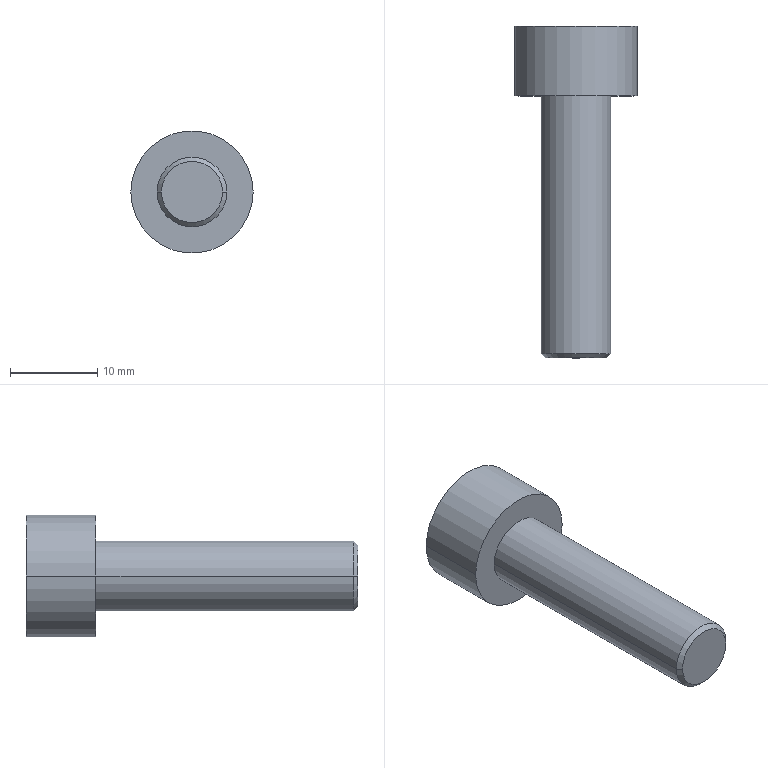Component | SolidWorks | M8x30HexSocketCap-2 | 1 solid | 16 faces | box 14 x 38 x 14 mm | volume 2553 mm3 | plane 10 | cylinder 4 | cone 2 | commonest cylinder face diameters 8 x2 14 x2 | material #45
build123d program:
from build123d import *

# Parameters (mm, degrees)
CUT_EXTRUDE1_DEPTH = 5.5


with BuildPart() as part:
    # Sketch1 → Revolve1 (revolve)
    with BuildSketch(Plane(origin=(0, 0, 0), x_dir=(1, 0, 0), z_dir=(0, 1, 0)), mode=Mode.PRIVATE) as revolve1_sk:
        Polygon((0, 38), (-7, 38), (-7, 30), (-4, 30), (-4, 0.5), (-3.5, 0), (0, 0), align=None)
    revolve(revolve1_sk.sketch.rotate(Axis((0, 0, 0), (0, 0, -1)), 180), axis=Axis((0, 0, 0), (0, 0, -1)))

    # Sketch2 → Cut-Extrude1 (cut)
    with BuildSketch(Plane(origin=(0, 0, -38), x_dir=(-1, 0, 0), z_dir=(0, 0, -1))):
        Polygon((0, 3.58), (-3.1, 1.79), (-3.1, -1.79), (0, -3.58), (3.1, -1.79), (3.1, 1.79), align=None)
    extrude(amount=-CUT_EXTRUDE1_DEPTH, mode=Mode.SUBTRACT)


solid = part.part

# Placed as in the assembly
solid = solid.moved(Location((7, -20, -15), (90, 0, 0)))
STEP:
#1=CARTESIAN_POINT('',(0.4134,-0.7874,-0.5906));
#2=VERTEX_POINT('',#1);
#3=CARTESIAN_POINT('',(0.1378,-0.7874,-0.5906));
#4=VERTEX_POINT('',#3);
#5=CARTESIAN_POINT('',(0.2756,-0.7874,-0.5906));
#6=DIRECTION('',(0.,-1.,0.));
#7=DIRECTION('',(1.,0.,0.));
#8=AXIS2_PLACEMENT_3D('',#5,#6,#7);
#9=CIRCLE('',#8,0.1378);
#10=EDGE_CURVE('',#2,#4,#9,.T.);
#11=ORIENTED_EDGE('',*,*,#10,.F.);
#12=CARTESIAN_POINT('',(0.4331,-0.7677,-0.5906));
#13=VERTEX_POINT('',#12);
#14=CARTESIAN_POINT('',(0.4331,-0.7677,-0.5906));
#15=DIRECTION('',(0.7071,0.7071,0.));
#16=VECTOR('',#15,39.37);
#17=LINE('',#14,#16);
#18=EDGE_CURVE('',#2,#13,#17,.T.);
#19=ORIENTED_EDGE('',*,*,#18,.T.);
#20=CARTESIAN_POINT('',(0.1181,-0.7677,-0.5906));
#21=VERTEX_POINT('',#20);
#22=CARTESIAN_POINT('',(0.2756,-0.7677,-0.5906));
#23=DIRECTION('',(0.,-1.,0.));
#24=DIRECTION('',(1.,0.,0.));
#25=AXIS2_PLACEMENT_3D('',#22,#23,#24);
#26=CIRCLE('',#25,0.1575);
#27=EDGE_CURVE('',#13,#21,#26,.T.);
#28=ORIENTED_EDGE('',*,*,#27,.T.);
#29=CARTESIAN_POINT('',(0.1181,-0.7677,-0.5906));
#30=DIRECTION('',(-0.7071,0.7071,0.));
#31=VECTOR('',#30,39.37);
#32=LINE('',#29,#31);
#33=EDGE_CURVE('',#4,#21,#32,.T.);
#34=ORIENTED_EDGE('',*,*,#33,.F.);
#35=EDGE_LOOP('',(#11,#19,#28,#34));
#36=FACE_OUTER_BOUND('',#35,.T.);
#37=CARTESIAN_POINT('',(0.2756,-0.7677,-0.5906));
#38=DIRECTION('',(0.,1.,0.));
#39=DIRECTION('',(-1.,0.,0.));
#40=AXIS2_PLACEMENT_3D('',#37,#38,#39);
#41=CONICAL_SURFACE('',#40,0.1575,0.7854);
#42=ADVANCED_FACE('',(#36),#41,.T.);
#43=CARTESIAN_POINT('',(0.4331,0.3937,-0.5906));
#44=VERTEX_POINT('',#43);
#45=CARTESIAN_POINT('',(0.1181,0.3937,-0.5906));
#46=VERTEX_POINT('',#45);
#47=CARTESIAN_POINT('',(0.2756,0.3937,-0.5906));
#48=DIRECTION('',(0.,-1.,0.));
#49=DIRECTION('',(1.,0.,0.));
#50=AXIS2_PLACEMENT_3D('',#47,#48,#49);
#51=CIRCLE('',#50,0.1575);
#52=EDGE_CURVE('',#44,#46,#51,.T.);
#53=ORIENTED_EDGE('',*,*,#52,.T.);
#54=CARTESIAN_POINT('',(0.1181,-0.7874,-0.5906));
#55=DIRECTION('',(0.,-1.,0.));
#56=VECTOR('',#55,39.37);
#57=LINE('',#54,#56);
#58=EDGE_CURVE('',#46,#21,#57,.T.);
#59=ORIENTED_EDGE('',*,*,#58,.T.);
#60=ORIENTED_EDGE('',*,*,#27,.F.);
#61=CARTESIAN_POINT('',(0.4331,-0.7874,-0.5906));
#62=DIRECTION('',(0.,-1.,0.));
#63=VECTOR('',#62,39.37);
#64=LINE('',#61,#63);
#65=EDGE_CURVE('',#44,#13,#64,.T.);
#66=ORIENTED_EDGE('',*,*,#65,.F.);
#67=EDGE_LOOP('',(#53,#59,#60,#66));
#68=FACE_OUTER_BOUND('',#67,.T.);
#69=CARTESIAN_POINT('',(0.2756,-0.7874,-0.5906));
#70=DIRECTION('',(0.,-1.,0.));
#71=DIRECTION('',(1.,0.,0.));
#72=AXIS2_PLACEMENT_3D('',#69,#70,#71);
#73=CYLINDRICAL_SURFACE('',#72,0.1575);
#74=ADVANCED_FACE('',(#68),#73,.T.);
#75=CARTESIAN_POINT('',(0.5512,0.7087,-0.5906));
#76=VERTEX_POINT('',#75);
#77=CARTESIAN_POINT('',(-0.,0.7087,-0.5906));
#78=VERTEX_POINT('',#77);
#79=CARTESIAN_POINT('',(0.2756,0.7087,-0.5906));
#80=DIRECTION('',(0.,-1.,0.));
#81=DIRECTION('',(1.,0.,0.));
#82=AXIS2_PLACEMENT_3D('',#79,#80,#81);
#83=CIRCLE('',#82,0.2756);
#84=EDGE_CURVE('',#76,#78,#83,.T.);
#85=ORIENTED_EDGE('',*,*,#84,.T.);
#86=CARTESIAN_POINT('',(-0.,0.3937,-0.5906));
#87=VERTEX_POINT('',#86);
#88=CARTESIAN_POINT('',(-0.,-0.7874,-0.5906));
#89=DIRECTION('',(0.,-1.,0.));
#90=VECTOR('',#89,39.37);
#91=LINE('',#88,#90);
#92=EDGE_CURVE('',#78,#87,#91,.T.);
#93=ORIENTED_EDGE('',*,*,#92,.T.);
#94=CARTESIAN_POINT('',(0.5512,0.3937,-0.5906));
#95=VERTEX_POINT('',#94);
#96=CARTESIAN_POINT('',(0.2756,0.3937,-0.5906));
#97=DIRECTION('',(0.,-1.,0.));
#98=DIRECTION('',(1.,0.,0.));
#99=AXIS2_PLACEMENT_3D('',#96,#97,#98);
#100=CIRCLE('',#99,0.2756);
#101=EDGE_CURVE('',#95,#87,#100,.T.);
#102=ORIENTED_EDGE('',*,*,#101,.F.);
#103=CARTESIAN_POINT('',(0.5512,-0.7874,-0.5906));
#104=DIRECTION('',(0.,-1.,0.));
#105=VECTOR('',#104,39.37);
#106=LINE('',#103,#105);
#107=EDGE_CURVE('',#76,#95,#106,.T.);
#108=ORIENTED_EDGE('',*,*,#107,.F.);
#109=EDGE_LOOP('',(#85,#93,#102,#108));
#110=FACE_OUTER_BOUND('',#109,.T.);
#111=CARTESIAN_POINT('',(0.2756,-0.7874,-0.5906));
#112=DIRECTION('',(0.,-1.,0.));
#113=DIRECTION('',(1.,0.,0.));
#114=AXIS2_PLACEMENT_3D('',#111,#112,#113);
#115=CYLINDRICAL_SURFACE('',#114,0.2756);
#116=ADVANCED_FACE('',(#110),#115,.T.);
#117=CARTESIAN_POINT('',(0.2756,0.7087,-0.4496));
#118=VERTEX_POINT('',#117);
#119=CARTESIAN_POINT('',(0.3976,0.7087,-0.5201));
#120=VERTEX_POINT('',#119);
#121=CARTESIAN_POINT('',(0.2756,0.7087,-0.4496));
#122=DIRECTION('',(0.866,0.,-0.5));
#123=VECTOR('',#122,39.37);
#124=LINE('',#121,#123);
#125=EDGE_CURVE('',#118,#120,#124,.T.);
#126=ORIENTED_EDGE('',*,*,#125,.F.);
#127=CARTESIAN_POINT('',(0.1535,0.7087,-0.5201));
#128=VERTEX_POINT('',#127);
#129=CARTESIAN_POINT('',(0.1535,0.7087,-0.5201));
#130=DIRECTION('',(0.866,0.,0.5));
#131=VECTOR('',#130,39.37);
#132=LINE('',#129,#131);
#133=EDGE_CURVE('',#128,#118,#132,.T.);
#134=ORIENTED_EDGE('',*,*,#133,.F.);
#135=CARTESIAN_POINT('',(0.1535,0.7087,-0.661));
#136=VERTEX_POINT('',#135);
#137=CARTESIAN_POINT('',(0.1535,0.7087,-0.661));
#138=DIRECTION('',(0.,0.,1.));
#139=VECTOR('',#138,39.37);
#140=LINE('',#137,#139);
#141=EDGE_CURVE('',#136,#128,#140,.T.);
#142=ORIENTED_EDGE('',*,*,#141,.F.);
#143=CARTESIAN_POINT('',(0.2756,0.7087,-0.7315));
#144=VERTEX_POINT('',#143);
#145=CARTESIAN_POINT('',(0.2756,0.7087,-0.7315));
#146=DIRECTION('',(-0.866,0.,0.5));
#147=VECTOR('',#146,39.37);
#148=LINE('',#145,#147);
#149=EDGE_CURVE('',#144,#136,#148,.T.);
#150=ORIENTED_EDGE('',*,*,#149,.F.);
#151=CARTESIAN_POINT('',(0.3976,0.7087,-0.661));
#152=VERTEX_POINT('',#151);
#153=CARTESIAN_POINT('',(0.3976,0.7087,-0.661));
#154=DIRECTION('',(-0.866,0.,-0.5));
#155=VECTOR('',#154,39.37);
#156=LINE('',#153,#155);
#157=EDGE_CURVE('',#152,#144,#156,.T.);
#158=ORIENTED_EDGE('',*,*,#157,.F.);
#159=CARTESIAN_POINT('',(0.3976,0.7087,-0.5201));
#160=DIRECTION('',(0.,0.,-1.));
#161=VECTOR('',#160,39.37);
#162=LINE('',#159,#161);
#163=EDGE_CURVE('',#120,#152,#162,.T.);
#164=ORIENTED_EDGE('',*,*,#163,.F.);
#165=EDGE_LOOP('',(#126,#134,#142,#150,#158,#164));
#166=FACE_BOUND('',#165,.T.);
#167=ORIENTED_EDGE('',*,*,#84,.F.);
#168=CARTESIAN_POINT('',(0.2756,0.7087,-0.5906));
#169=DIRECTION('',(0.,-1.,0.));
#170=DIRECTION('',(1.,0.,0.));
#171=AXIS2_PLACEMENT_3D('',#168,#169,#170);
#172=CIRCLE('',#171,0.2756);
#173=EDGE_CURVE('',#78,#76,#172,.T.);
#174=ORIENTED_EDGE('',*,*,#173,.F.);
#175=EDGE_LOOP('',(#167,#174));
#176=FACE_OUTER_BOUND('',#175,.T.);
#177=CARTESIAN_POINT('',(0.2756,0.7087,-0.5906));
#178=DIRECTION('',(0.,-1.,0.));
#179=DIRECTION('',(1.,0.,0.));
#180=AXIS2_PLACEMENT_3D('',#177,#178,#179);
#181=PLANE('',#180);
#182=ADVANCED_FACE('',(#166,#176),#181,.F.);
#183=ORIENTED_EDGE('',*,*,#92,.F.);
#184=ORIENTED_EDGE('',*,*,#173,.T.);
#185=ORIENTED_EDGE('',*,*,#107,.T.);
#186=CARTESIAN_POINT('',(0.2756,0.3937,-0.5906));
#187=DIRECTION('',(0.,-1.,0.));
#188=DIRECTION('',(1.,0.,0.));
#189=AXIS2_PLACEMENT_3D('',#186,#187,#188);
#190=CIRCLE('',#189,0.2756);
#191=EDGE_CURVE('',#87,#95,#190,.T.);
#192=ORIENTED_EDGE('',*,*,#191,.F.);
#193=EDGE_LOOP('',(#183,#184,#185,#192));
#194=FACE_OUTER_BOUND('',#193,.T.);
#195=CARTESIAN_POINT('',(0.2756,-0.7874,-0.5906));
#196=DIRECTION('',(0.,-1.,0.));
#197=DIRECTION('',(1.,0.,0.));
#198=AXIS2_PLACEMENT_3D('',#195,#196,#197);
#199=CYLINDRICAL_SURFACE('',#198,0.2756);
#200=ADVANCED_FACE('',(#194),#199,.T.);
#201=ORIENTED_EDGE('',*,*,#52,.F.);
#202=CARTESIAN_POINT('',(0.2756,0.3937,-0.5906));
#203=DIRECTION('',(0.,-1.,0.));
#204=DIRECTION('',(1.,0.,0.));
#205=AXIS2_PLACEMENT_3D('',#202,#203,#204);
#206=CIRCLE('',#205,0.1575);
#207=EDGE_CURVE('',#46,#44,#206,.T.);
#208=ORIENTED_EDGE('',*,*,#207,.F.);
#209=EDGE_LOOP('',(#201,#208));
#210=FACE_BOUND('',#209,.T.);
#211=ORIENTED_EDGE('',*,*,#101,.T.);
#212=ORIENTED_EDGE('',*,*,#191,.T.);
#213=EDGE_LOOP('',(#211,#212));
#214=FACE_OUTER_BOUND('',#213,.T.);
#215=CARTESIAN_POINT('',(-0.,0.3937,-0.5906));
#216=DIRECTION('',(0.,1.,0.));
#217=DIRECTION('',(-1.,0.,0.));
#218=AXIS2_PLACEMENT_3D('',#215,#216,#217);
#219=PLANE('',#218);
#220=ADVANCED_FACE('',(#210,#214),#219,.F.);
#221=ORIENTED_EDGE('',*,*,#58,.F.);
#222=ORIENTED_EDGE('',*,*,#207,.T.);
#223=ORIENTED_EDGE('',*,*,#65,.T.);
#224=CARTESIAN_POINT('',(0.2756,-0.7677,-0.5906));
#225=DIRECTION('',(0.,-1.,0.));
#226=DIRECTION('',(1.,0.,0.));
#227=AXIS2_PLACEMENT_3D('',#224,#225,#226);
#228=CIRCLE('',#227,0.1575);
#229=EDGE_CURVE('',#21,#13,#228,.T.);
#230=ORIENTED_EDGE('',*,*,#229,.F.);
#231=EDGE_LOOP('',(#221,#222,#223,#230));
#232=FACE_OUTER_BOUND('',#231,.T.);
#233=CARTESIAN_POINT('',(0.2756,-0.7874,-0.5906));
#234=DIRECTION('',(0.,-1.,0.));
#235=DIRECTION('',(1.,0.,0.));
#236=AXIS2_PLACEMENT_3D('',#233,#234,#235);
#237=CYLINDRICAL_SURFACE('',#236,0.1575);
#238=ADVANCED_FACE('',(#232),#237,.T.);
#239=ORIENTED_EDGE('',*,*,#18,.F.);
#240=CARTESIAN_POINT('',(0.2756,-0.7874,-0.5906));
#241=DIRECTION('',(0.,-1.,0.));
#242=DIRECTION('',(1.,0.,0.));
#243=AXIS2_PLACEMENT_3D('',#240,#241,#242);
#244=CIRCLE('',#243,0.1378);
#245=EDGE_CURVE('',#4,#2,#244,.T.);
#246=ORIENTED_EDGE('',*,*,#245,.F.);
#247=ORIENTED_EDGE('',*,*,#33,.T.);
#248=ORIENTED_EDGE('',*,*,#229,.T.);
#249=EDGE_LOOP('',(#239,#246,#247,#248));
#250=FACE_OUTER_BOUND('',#249,.T.);
#251=CARTESIAN_POINT('',(0.2756,-0.7677,-0.5906));
#252=DIRECTION('',(0.,1.,0.));
#253=DIRECTION('',(-1.,0.,0.));
#254=AXIS2_PLACEMENT_3D('',#251,#252,#253);
#255=CONICAL_SURFACE('',#254,0.1575,0.7854);
#256=ADVANCED_FACE('',(#250),#255,.T.);
#257=ORIENTED_EDGE('',*,*,#245,.T.);
#258=ORIENTED_EDGE('',*,*,#10,.T.);
#259=EDGE_LOOP('',(#257,#258));
#260=FACE_OUTER_BOUND('',#259,.T.);
#261=CARTESIAN_POINT('',(0.1378,-0.7874,-0.5906));
#262=DIRECTION('',(0.,1.,0.));
#263=DIRECTION('',(-1.,0.,0.));
#264=AXIS2_PLACEMENT_3D('',#261,#262,#263);
#265=PLANE('',#264);
#266=ADVANCED_FACE('',(#260),#265,.F.);
#267=ORIENTED_EDGE('',*,*,#133,.T.);
#268=CARTESIAN_POINT('',(0.2756,0.4921,-0.4496));
#269=VERTEX_POINT('',#268);
#270=CARTESIAN_POINT('',(0.2756,0.4921,-0.4496));
#271=DIRECTION('',(0.,1.,0.));
#272=VECTOR('',#271,39.37);
#273=LINE('',#270,#272);
#274=EDGE_CURVE('',#269,#118,#273,.T.);
#275=ORIENTED_EDGE('',*,*,#274,.F.);
#276=CARTESIAN_POINT('',(0.1535,0.4921,-0.5201));
#277=VERTEX_POINT('',#276);
#278=CARTESIAN_POINT('',(0.1535,0.4921,-0.5201));
#279=DIRECTION('',(0.866,0.,0.5));
#280=VECTOR('',#279,39.37);
#281=LINE('',#278,#280);
#282=EDGE_CURVE('',#277,#269,#281,.T.);
#283=ORIENTED_EDGE('',*,*,#282,.F.);
#284=CARTESIAN_POINT('',(0.1535,0.4921,-0.5201));
#285=DIRECTION('',(0.,1.,0.));
#286=VECTOR('',#285,39.37);
#287=LINE('',#284,#286);
#288=EDGE_CURVE('',#277,#128,#287,.T.);
#289=ORIENTED_EDGE('',*,*,#288,.T.);
#290=EDGE_LOOP('',(#267,#275,#283,#289));
#291=FACE_OUTER_BOUND('',#290,.T.);
#292=CARTESIAN_POINT('',(0.1535,0.4921,-0.5201));
#293=DIRECTION('',(-0.5,0.,0.866));
#294=DIRECTION('',(-0.866,0.,-0.5));
#295=AXIS2_PLACEMENT_3D('',#292,#293,#294);
#296=PLANE('',#295);
#297=ADVANCED_FACE('',(#291),#296,.F.);
#298=ORIENTED_EDGE('',*,*,#141,.T.);
#299=ORIENTED_EDGE('',*,*,#288,.F.);
#300=CARTESIAN_POINT('',(0.1535,0.4921,-0.661));
#301=VERTEX_POINT('',#300);
#302=CARTESIAN_POINT('',(0.1535,0.4921,-0.661));
#303=DIRECTION('',(0.,0.,1.));
#304=VECTOR('',#303,39.37);
#305=LINE('',#302,#304);
#306=EDGE_CURVE('',#301,#277,#305,.T.);
#307=ORIENTED_EDGE('',*,*,#306,.F.);
#308=CARTESIAN_POINT('',(0.1535,0.4921,-0.661));
#309=DIRECTION('',(0.,1.,0.));
#310=VECTOR('',#309,39.37);
#311=LINE('',#308,#310);
#312=EDGE_CURVE('',#301,#136,#311,.T.);
#313=ORIENTED_EDGE('',*,*,#312,.T.);
#314=EDGE_LOOP('',(#298,#299,#307,#313));
#315=FACE_OUTER_BOUND('',#314,.T.);
#316=CARTESIAN_POINT('',(0.1535,0.4921,-0.661));
#317=DIRECTION('',(-1.,0.,0.));
#318=DIRECTION('',(-0.,0.,-1.));
#319=AXIS2_PLACEMENT_3D('',#316,#317,#318);
#320=PLANE('',#319);
#321=ADVANCED_FACE('',(#315),#320,.F.);
#322=ORIENTED_EDGE('',*,*,#149,.T.);
#323=ORIENTED_EDGE('',*,*,#312,.F.);
#324=CARTESIAN_POINT('',(0.2756,0.4921,-0.7315));
#325=VERTEX_POINT('',#324);
#326=CARTESIAN_POINT('',(0.2756,0.4921,-0.7315));
#327=DIRECTION('',(-0.866,0.,0.5));
#328=VECTOR('',#327,39.37);
#329=LINE('',#326,#328);
#330=EDGE_CURVE('',#325,#301,#329,.T.);
#331=ORIENTED_EDGE('',*,*,#330,.F.);
#332=CARTESIAN_POINT('',(0.2756,0.4921,-0.7315));
#333=DIRECTION('',(0.,1.,0.));
#334=VECTOR('',#333,39.37);
#335=LINE('',#332,#334);
#336=EDGE_CURVE('',#325,#144,#335,.T.);
#337=ORIENTED_EDGE('',*,*,#336,.T.);
#338=EDGE_LOOP('',(#322,#323,#331,#337));
#339=FACE_OUTER_BOUND('',#338,.T.);
#340=CARTESIAN_POINT('',(0.2756,0.4921,-0.7315));
#341=DIRECTION('',(-0.5,0.,-0.866));
#342=DIRECTION('',(0.866,0.,-0.5));
#343=AXIS2_PLACEMENT_3D('',#340,#341,#342);
#344=PLANE('',#343);
#345=ADVANCED_FACE('',(#339),#344,.F.);
#346=ORIENTED_EDGE('',*,*,#157,.T.);
#347=ORIENTED_EDGE('',*,*,#336,.F.);
#348=CARTESIAN_POINT('',(0.3976,0.4921,-0.661));
#349=VERTEX_POINT('',#348);
#350=CARTESIAN_POINT('',(0.3976,0.4921,-0.661));
#351=DIRECTION('',(-0.866,0.,-0.5));
#352=VECTOR('',#351,39.37);
#353=LINE('',#350,#352);
#354=EDGE_CURVE('',#349,#325,#353,.T.);
#355=ORIENTED_EDGE('',*,*,#354,.F.);
#356=CARTESIAN_POINT('',(0.3976,0.4921,-0.661));
#357=DIRECTION('',(0.,1.,0.));
#358=VECTOR('',#357,39.37);
#359=LINE('',#356,#358);
#360=EDGE_CURVE('',#349,#152,#359,.T.);
#361=ORIENTED_EDGE('',*,*,#360,.T.);
#362=EDGE_LOOP('',(#346,#347,#355,#361));
#363=FACE_OUTER_BOUND('',#362,.T.);
#364=CARTESIAN_POINT('',(0.3976,0.4921,-0.661));
#365=DIRECTION('',(0.5,0.,-0.866));
#366=DIRECTION('',(0.866,0.,0.5));
#367=AXIS2_PLACEMENT_3D('',#364,#365,#366);
#368=PLANE('',#367);
#369=ADVANCED_FACE('',(#363),#368,.F.);
#370=ORIENTED_EDGE('',*,*,#163,.T.);
#371=ORIENTED_EDGE('',*,*,#360,.F.);
#372=CARTESIAN_POINT('',(0.3976,0.4921,-0.5201));
#373=VERTEX_POINT('',#372);
#374=CARTESIAN_POINT('',(0.3976,0.4921,-0.5201));
#375=DIRECTION('',(0.,0.,-1.));
#376=VECTOR('',#375,39.37);
#377=LINE('',#374,#376);
#378=EDGE_CURVE('',#373,#349,#377,.T.);
#379=ORIENTED_EDGE('',*,*,#378,.F.);
#380=CARTESIAN_POINT('',(0.3976,0.4921,-0.5201));
#381=DIRECTION('',(0.,1.,0.));
#382=VECTOR('',#381,39.37);
#383=LINE('',#380,#382);
#384=EDGE_CURVE('',#373,#120,#383,.T.);
#385=ORIENTED_EDGE('',*,*,#384,.T.);
#386=EDGE_LOOP('',(#370,#371,#379,#385));
#387=FACE_OUTER_BOUND('',#386,.T.);
#388=CARTESIAN_POINT('',(0.3976,0.4921,-0.5201));
#389=DIRECTION('',(1.,0.,0.));
#390=DIRECTION('',(0.,1.,0.));
#391=AXIS2_PLACEMENT_3D('',#388,#389,#390);
#392=PLANE('',#391);
#393=ADVANCED_FACE('',(#387),#392,.F.);
#394=ORIENTED_EDGE('',*,*,#125,.T.);
#395=ORIENTED_EDGE('',*,*,#384,.F.);
#396=CARTESIAN_POINT('',(0.2756,0.4921,-0.4496));
#397=DIRECTION('',(0.866,0.,-0.5));
#398=VECTOR('',#397,39.37);
#399=LINE('',#396,#398);
#400=EDGE_CURVE('',#269,#373,#399,.T.);
#401=ORIENTED_EDGE('',*,*,#400,.F.);
#402=ORIENTED_EDGE('',*,*,#274,.T.);
#403=EDGE_LOOP('',(#394,#395,#401,#402));
#404=FACE_OUTER_BOUND('',#403,.T.);
#405=CARTESIAN_POINT('',(0.2756,0.4921,-0.4496));
#406=DIRECTION('',(0.5,0.,0.866));
#407=DIRECTION('',(-0.866,0.,0.5));
#408=AXIS2_PLACEMENT_3D('',#405,#406,#407);
#409=PLANE('',#408);
#410=ADVANCED_FACE('',(#404),#409,.F.);
#411=ORIENTED_EDGE('',*,*,#282,.T.);
#412=ORIENTED_EDGE('',*,*,#400,.T.);
#413=ORIENTED_EDGE('',*,*,#378,.T.);
#414=ORIENTED_EDGE('',*,*,#354,.T.);
#415=ORIENTED_EDGE('',*,*,#330,.T.);
#416=ORIENTED_EDGE('',*,*,#306,.T.);
#417=EDGE_LOOP('',(#411,#412,#413,#414,#415,#416));
#418=FACE_OUTER_BOUND('',#417,.T.);
#419=CARTESIAN_POINT('',(0.2756,0.4921,-0.5906));
#420=DIRECTION('',(0.,1.,0.));
#421=DIRECTION('',(-1.,0.,0.));
#422=AXIS2_PLACEMENT_3D('',#419,#420,#421);
#423=PLANE('',#422);
#424=ADVANCED_FACE('',(#418),#423,.T.);
#425=CLOSED_SHELL('',(#42,#74,#116,#182,#200,#220,#238,#256,#266,#297,#321,#345,#369,#393,#410,#424));
#426=MANIFOLD_SOLID_BREP('',#425);
#427=CARTESIAN_POINT('',(0.,0.,0.));
#428=DIRECTION('',(0.,0.,1.));
#429=DIRECTION('',(1.,0.,0.));
#430=AXIS2_PLACEMENT_3D('',#427,#428,#429);
#431=(LENGTH_UNIT()NAMED_UNIT(*)SI_UNIT($,.METRE.));
#432=LENGTH_MEASURE_WITH_UNIT(LENGTH_MEASURE(0.0254),#431);
#433=DIMENSIONAL_EXPONENTS(1.,0.,0.,0.,0.,0.,0.);
#434=(CONVERSION_BASED_UNIT('',#432)LENGTH_UNIT()NAMED_UNIT(#433));
#435=UNCERTAINTY_MEASURE_WITH_UNIT(LENGTH_MEASURE(0.00001),#434,'','');
#436=(NAMED_UNIT(*)PLANE_ANGLE_UNIT()SI_UNIT($,.RADIAN.));
#437=(NAMED_UNIT(*)SI_UNIT($,.STERADIAN.)SOLID_ANGLE_UNIT());
#438=(GEOMETRIC_REPRESENTATION_CONTEXT(3)GLOBAL_UNCERTAINTY_ASSIGNED_CONTEXT((#435))GLOBAL_UNIT_ASSIGNED_CONTEXT((#434,#436,#437))REPRESENTATION_CONTEXT('',''));
#439=ADVANCED_BREP_SHAPE_REPRESENTATION('',(#426,#430),#438);
#440=COLOUR_RGB('',0.7922,0.8196,0.9333);
#441=FILL_AREA_STYLE_COLOUR('',#440);
#442=FILL_AREA_STYLE('',(#441));
#443=SURFACE_STYLE_FILL_AREA(#442);
#444=SURFACE_SIDE_STYLE('',(#443));
#445=SURFACE_STYLE_USAGE(.BOTH.,#444);
#446=PRESENTATION_STYLE_ASSIGNMENT((#445));
#447=STYLED_ITEM('',(#446),#426);
#448=(LENGTH_UNIT()NAMED_UNIT(*)SI_UNIT($,.METRE.));
#449=LENGTH_MEASURE_WITH_UNIT(LENGTH_MEASURE(0.0254),#448);
#450=DIMENSIONAL_EXPONENTS(1.,0.,0.,0.,0.,0.,0.);
#451=(CONVERSION_BASED_UNIT('',#449)LENGTH_UNIT()NAMED_UNIT(#450));
#452=UNCERTAINTY_MEASURE_WITH_UNIT(LENGTH_MEASURE(0.00001),#451,'','');
#453=(NAMED_UNIT(*)PLANE_ANGLE_UNIT()SI_UNIT($,.RADIAN.));
#454=(NAMED_UNIT(*)SI_UNIT($,.STERADIAN.)SOLID_ANGLE_UNIT());
#455=(GEOMETRIC_REPRESENTATION_CONTEXT(3)GLOBAL_UNCERTAINTY_ASSIGNED_CONTEXT((#452))GLOBAL_UNIT_ASSIGNED_CONTEXT((#451,#453,#454))REPRESENTATION_CONTEXT('',''));
#456=MECHANICAL_DESIGN_GEOMETRIC_PRESENTATION_REPRESENTATION('',(#447),#455);
#457=PRESENTATION_LAYER_ASSIGNMENT('','',(#447));